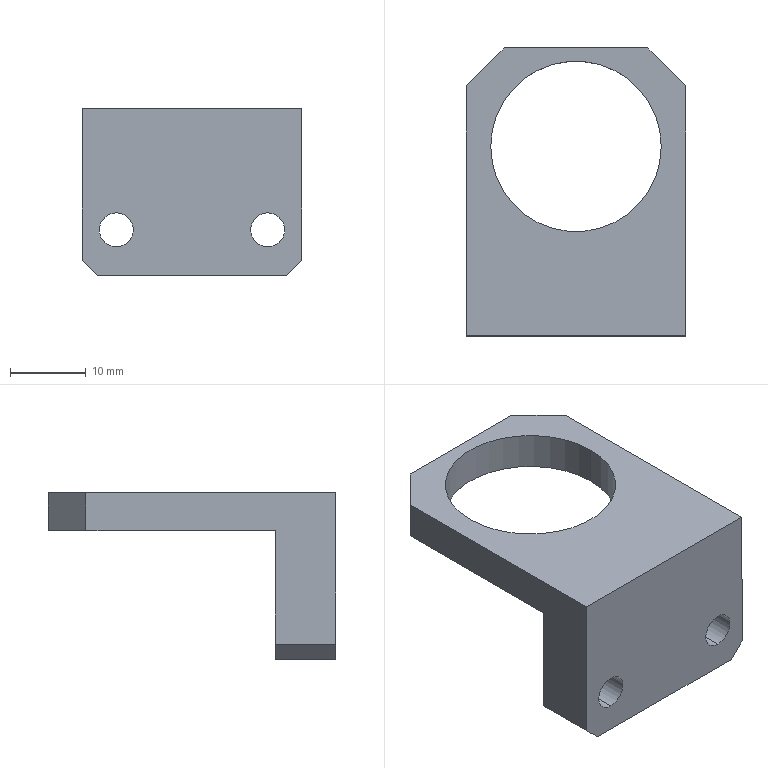Component | SolidWorks | F01AE00111-A2000-21TopEdgeAssembly-1_F01AE00111-A2055-1 | 1 solid | 18 faces | box 29 x 38 x 22 mm | volume 7054 mm3 | plane 12 | cylinder 6 | commonest cylinder face diameters 4.5 x4 22.5 x2
build123d program:
from build123d import *

# Parameters (mm, degrees)
SKETCH1_W           = 29
SKETCH1_H           = 38
BOSS_EXTRUDE1_DEPTH = 8
SKETCH2_W           = 22
SKETCH2_H           = 8
BOSS_EXTRUDE2_DEPTH = 29
SKETCH3_R           = 11.25
CUT_EXTRUDE1_DEPTH  = 12
CHAMFER1_SIZE       = 5
CHAMFER2_SIZE       = 2
SKETCH5_R           = 2.25
CUT_EXTRUDE3_DEPTH  = 12
SKETCH6_W           = 34.275
SKETCH6_H           = 35.36
CUT_EXTRUDE4_DEPTH  = 3


with BuildPart() as part:
    # Sketch1 → Boss-Extrude1 (new body)
    with BuildSketch(Plane.XY):
        Rectangle(SKETCH1_W, SKETCH1_H)
    extrude(amount=BOSS_EXTRUDE1_DEPTH)

    # Sketch2 → Boss-Extrude2 (add)
    with BuildSketch(Plane(origin=(14.5, 0, 0), x_dir=(0, 0, -1), z_dir=(1, 0, 0))):
        with Locations((3, -15)):
            Rectangle(SKETCH2_W, SKETCH2_H)
    extrude(amount=-BOSS_EXTRUDE2_DEPTH)

    # Sketch3 → Cut-Extrude1 (cut)
    with BuildSketch(Plane(origin=(0, 0, 0), x_dir=(-1, 0, 0), z_dir=(0, 0, -1))):
        with Locations((0, 6)):
            Circle(SKETCH3_R)
    extrude(amount=-CUT_EXTRUDE1_DEPTH, mode=Mode.SUBTRACT)

    # Chamfer1
    chamfer1_edges = [part.edges().sort_by_distance(p)[0] for p in [
        (-14.5, 19, 4),
        (14.5, 19, 4),
    ]]
    chamfer(chamfer1_edges, length=CHAMFER1_SIZE)

    # Chamfer2
    chamfer2_edges = [part.edges().sort_by_distance(p)[0] for p in [
        (14.5, -15, -14),
        (-14.5, -15, -14),
    ]]
    chamfer(chamfer2_edges, length=CHAMFER2_SIZE)

    # Sketch5 → Cut-Extrude3 (cut)
    with BuildSketch(Plane(origin=(0, -11, 0), x_dir=(1, 0, 0), z_dir=(0, 1, 0))):
        with Locations(Location((-10, 8, 0), (0, 0, 270))):
            Circle(SKETCH5_R)
        with Locations(Location((10, 8, 0), (0, 0, 270))):
            Circle(SKETCH5_R)
    extrude(amount=-CUT_EXTRUDE3_DEPTH, mode=Mode.SUBTRACT)

    # Sketch6 → Cut-Extrude4 (cut)
    with BuildSketch(Plane(origin=(0, 0, 0), x_dir=(-1, 0, 0), z_dir=(0, 0, -1))):
        with Locations((2.637, 6.68)):
            Rectangle(SKETCH6_W, SKETCH6_H)
    extrude(amount=-CUT_EXTRUDE4_DEPTH, mode=Mode.SUBTRACT)


solid = part.part

# Placed as in the assembly
solid = solid.moved(Location((-109.352, 76.548, -339.975), (0, 0, 0)))
STEP:
#1=CARTESIAN_POINT('',(-3.911,2.266,-13.788));
#2=VERTEX_POINT('',#1);
#3=CARTESIAN_POINT('',(-3.911,2.266,-13.611));
#4=VERTEX_POINT('',#3);
#5=CARTESIAN_POINT('',(-3.911,2.266,-13.7));
#6=DIRECTION('',(0.,1.,0.));
#7=DIRECTION('',(0.,0.,1.));
#8=AXIS2_PLACEMENT_3D('',#5,#6,#7);
#9=CIRCLE('',#8,0.08858);
#10=EDGE_CURVE('',#2,#4,#9,.T.);
#11=ORIENTED_EDGE('',*,*,#10,.F.);
#12=CARTESIAN_POINT('',(-3.911,2.581,-13.788));
#13=VERTEX_POINT('',#12);
#14=CARTESIAN_POINT('',(-3.911,2.108,-13.788));
#15=DIRECTION('',(0.,1.,0.));
#16=VECTOR('',#15,39.37);
#17=LINE('',#14,#16);
#18=EDGE_CURVE('',#2,#13,#17,.T.);
#19=ORIENTED_EDGE('',*,*,#18,.T.);
#20=CARTESIAN_POINT('',(-3.911,2.581,-13.611));
#21=VERTEX_POINT('',#20);
#22=CARTESIAN_POINT('',(-3.911,2.581,-13.7));
#23=DIRECTION('',(0.,1.,0.));
#24=DIRECTION('',(0.,0.,1.));
#25=AXIS2_PLACEMENT_3D('',#22,#23,#24);
#26=CIRCLE('',#25,0.08858);
#27=EDGE_CURVE('',#13,#21,#26,.T.);
#28=ORIENTED_EDGE('',*,*,#27,.T.);
#29=CARTESIAN_POINT('',(-3.911,2.108,-13.611));
#30=DIRECTION('',(0.,1.,0.));
#31=VECTOR('',#30,39.37);
#32=LINE('',#29,#31);
#33=EDGE_CURVE('',#4,#21,#32,.T.);
#34=ORIENTED_EDGE('',*,*,#33,.F.);
#35=EDGE_LOOP('',(#11,#19,#28,#34));
#36=FACE_OUTER_BOUND('',#35,.T.);
#37=CARTESIAN_POINT('',(-3.911,2.108,-13.7));
#38=DIRECTION('',(0.,1.,0.));
#39=DIRECTION('',(0.,0.,1.));
#40=AXIS2_PLACEMENT_3D('',#37,#38,#39);
#41=CYLINDRICAL_SURFACE('',#40,0.08858);
#42=ADVANCED_FACE('',(#36),#41,.F.);
#43=CARTESIAN_POINT('',(-4.699,2.266,-13.788));
#44=VERTEX_POINT('',#43);
#45=CARTESIAN_POINT('',(-4.699,2.266,-13.611));
#46=VERTEX_POINT('',#45);
#47=CARTESIAN_POINT('',(-4.699,2.266,-13.7));
#48=DIRECTION('',(0.,1.,0.));
#49=DIRECTION('',(0.,0.,1.));
#50=AXIS2_PLACEMENT_3D('',#47,#48,#49);
#51=CIRCLE('',#50,0.08858);
#52=EDGE_CURVE('',#44,#46,#51,.T.);
#53=ORIENTED_EDGE('',*,*,#52,.F.);
#54=CARTESIAN_POINT('',(-4.699,2.581,-13.788));
#55=VERTEX_POINT('',#54);
#56=CARTESIAN_POINT('',(-4.699,2.108,-13.788));
#57=DIRECTION('',(0.,1.,0.));
#58=VECTOR('',#57,39.37);
#59=LINE('',#56,#58);
#60=EDGE_CURVE('',#44,#55,#59,.T.);
#61=ORIENTED_EDGE('',*,*,#60,.T.);
#62=CARTESIAN_POINT('',(-4.699,2.581,-13.611));
#63=VERTEX_POINT('',#62);
#64=CARTESIAN_POINT('',(-4.699,2.581,-13.7));
#65=DIRECTION('',(0.,1.,0.));
#66=DIRECTION('',(0.,0.,1.));
#67=AXIS2_PLACEMENT_3D('',#64,#65,#66);
#68=CIRCLE('',#67,0.08858);
#69=EDGE_CURVE('',#55,#63,#68,.T.);
#70=ORIENTED_EDGE('',*,*,#69,.T.);
#71=CARTESIAN_POINT('',(-4.699,2.108,-13.611));
#72=DIRECTION('',(0.,1.,0.));
#73=VECTOR('',#72,39.37);
#74=LINE('',#71,#73);
#75=EDGE_CURVE('',#46,#63,#74,.T.);
#76=ORIENTED_EDGE('',*,*,#75,.F.);
#77=EDGE_LOOP('',(#53,#61,#70,#76));
#78=FACE_OUTER_BOUND('',#77,.T.);
#79=CARTESIAN_POINT('',(-4.699,2.108,-13.7));
#80=DIRECTION('',(0.,1.,0.));
#81=DIRECTION('',(0.,0.,1.));
#82=AXIS2_PLACEMENT_3D('',#79,#80,#81);
#83=CYLINDRICAL_SURFACE('',#82,0.08858);
#84=ADVANCED_FACE('',(#78),#83,.F.);
#85=CARTESIAN_POINT('',(-3.862,3.25,-13.07));
#86=VERTEX_POINT('',#85);
#87=CARTESIAN_POINT('',(-4.748,3.25,-13.07));
#88=VERTEX_POINT('',#87);
#89=CARTESIAN_POINT('',(-4.305,3.25,-13.07));
#90=DIRECTION('',(0.,0.,-1.));
#91=DIRECTION('',(-1.,0.,0.));
#92=AXIS2_PLACEMENT_3D('',#89,#90,#91);
#93=CIRCLE('',#92,0.4429);
#94=EDGE_CURVE('',#86,#88,#93,.T.);
#95=ORIENTED_EDGE('',*,*,#94,.F.);
#96=CARTESIAN_POINT('',(-3.862,3.25,-13.267));
#97=VERTEX_POINT('',#96);
#98=CARTESIAN_POINT('',(-3.862,3.25,-12.912));
#99=DIRECTION('',(0.,0.,-1.));
#100=VECTOR('',#99,39.37);
#101=LINE('',#98,#100);
#102=EDGE_CURVE('',#86,#97,#101,.T.);
#103=ORIENTED_EDGE('',*,*,#102,.T.);
#104=CARTESIAN_POINT('',(-4.748,3.25,-13.267));
#105=VERTEX_POINT('',#104);
#106=CARTESIAN_POINT('',(-4.305,3.25,-13.267));
#107=DIRECTION('',(0.,0.,-1.));
#108=DIRECTION('',(1.,0.,0.));
#109=AXIS2_PLACEMENT_3D('',#106,#107,#108);
#110=CIRCLE('',#109,0.4429);
#111=EDGE_CURVE('',#97,#105,#110,.T.);
#112=ORIENTED_EDGE('',*,*,#111,.T.);
#113=CARTESIAN_POINT('',(-4.748,3.25,-12.912));
#114=DIRECTION('',(0.,0.,-1.));
#115=VECTOR('',#114,39.37);
#116=LINE('',#113,#115);
#117=EDGE_CURVE('',#88,#105,#116,.T.);
#118=ORIENTED_EDGE('',*,*,#117,.F.);
#119=EDGE_LOOP('',(#95,#103,#112,#118));
#120=FACE_OUTER_BOUND('',#119,.T.);
#121=CARTESIAN_POINT('',(-4.305,3.25,-12.912));
#122=DIRECTION('',(0.,0.,-1.));
#123=DIRECTION('',(-1.,0.,0.));
#124=AXIS2_PLACEMENT_3D('',#121,#122,#123);
#125=CYLINDRICAL_SURFACE('',#124,0.4429);
#126=ADVANCED_FACE('',(#120),#125,.F.);
#127=CARTESIAN_POINT('',(-3.734,2.581,-13.857));
#128=VERTEX_POINT('',#127);
#129=CARTESIAN_POINT('',(-3.734,2.581,-13.267));
#130=VERTEX_POINT('',#129);
#131=CARTESIAN_POINT('',(-3.734,2.581,-13.07));
#132=DIRECTION('',(0.,0.,1.));
#133=VECTOR('',#132,39.37);
#134=LINE('',#131,#133);
#135=EDGE_CURVE('',#128,#130,#134,.T.);
#136=ORIENTED_EDGE('',*,*,#135,.T.);
#137=CARTESIAN_POINT('',(-3.734,3.565,-13.267));
#138=VERTEX_POINT('',#137);
#139=CARTESIAN_POINT('',(-3.734,2.581,-13.267));
#140=DIRECTION('',(0.,-1.,0.));
#141=VECTOR('',#140,39.37);
#142=LINE('',#139,#141);
#143=EDGE_CURVE('',#138,#130,#142,.T.);
#144=ORIENTED_EDGE('',*,*,#143,.F.);
#145=CARTESIAN_POINT('',(-3.734,3.565,-13.07));
#146=VERTEX_POINT('',#145);
#147=CARTESIAN_POINT('',(-3.734,3.565,-13.07));
#148=DIRECTION('',(0.,0.,1.));
#149=VECTOR('',#148,39.37);
#150=LINE('',#147,#149);
#151=EDGE_CURVE('',#138,#146,#150,.T.);
#152=ORIENTED_EDGE('',*,*,#151,.T.);
#153=CARTESIAN_POINT('',(-3.734,2.266,-13.07));
#154=VERTEX_POINT('',#153);
#155=CARTESIAN_POINT('',(-3.734,2.266,-13.07));
#156=DIRECTION('',(0.,1.,0.));
#157=VECTOR('',#156,39.37);
#158=LINE('',#155,#157);
#159=EDGE_CURVE('',#154,#146,#158,.T.);
#160=ORIENTED_EDGE('',*,*,#159,.F.);
#161=CARTESIAN_POINT('',(-3.734,2.266,-13.857));
#162=VERTEX_POINT('',#161);
#163=CARTESIAN_POINT('',(-3.734,2.266,-13.07));
#164=DIRECTION('',(0.,0.,-1.));
#165=VECTOR('',#164,39.37);
#166=LINE('',#163,#165);
#167=EDGE_CURVE('',#154,#162,#166,.T.);
#168=ORIENTED_EDGE('',*,*,#167,.T.);
#169=CARTESIAN_POINT('',(-3.734,2.581,-13.857));
#170=DIRECTION('',(0.,1.,0.));
#171=VECTOR('',#170,39.37);
#172=LINE('',#169,#171);
#173=EDGE_CURVE('',#162,#128,#172,.T.);
#174=ORIENTED_EDGE('',*,*,#173,.T.);
#175=EDGE_LOOP('',(#136,#144,#152,#160,#168,#174));
#176=FACE_OUTER_BOUND('',#175,.T.);
#177=CARTESIAN_POINT('',(-3.734,2.266,-13.07));
#178=DIRECTION('',(-1.,0.,0.));
#179=DIRECTION('',(0.,0.,1.));
#180=AXIS2_PLACEMENT_3D('',#177,#178,#179);
#181=PLANE('',#180);
#182=ADVANCED_FACE('',(#176),#181,.F.);
#183=CARTESIAN_POINT('',(-3.931,3.762,-13.07));
#184=VERTEX_POINT('',#183);
#185=CARTESIAN_POINT('',(-3.931,3.762,-13.267));
#186=VERTEX_POINT('',#185);
#187=CARTESIAN_POINT('',(-3.931,3.762,-13.07));
#188=DIRECTION('',(0.,0.,-1.));
#189=VECTOR('',#188,39.37);
#190=LINE('',#187,#189);
#191=EDGE_CURVE('',#184,#186,#190,.T.);
#192=ORIENTED_EDGE('',*,*,#191,.T.);
#193=CARTESIAN_POINT('',(-4.679,3.762,-13.267));
#194=VERTEX_POINT('',#193);
#195=CARTESIAN_POINT('',(-4.876,3.762,-13.267));
#196=DIRECTION('',(-1.,0.,0.));
#197=VECTOR('',#196,39.37);
#198=LINE('',#195,#197);
#199=EDGE_CURVE('',#186,#194,#198,.T.);
#200=ORIENTED_EDGE('',*,*,#199,.T.);
#201=CARTESIAN_POINT('',(-4.679,3.762,-13.07));
#202=VERTEX_POINT('',#201);
#203=CARTESIAN_POINT('',(-4.679,3.762,-13.07));
#204=DIRECTION('',(0.,0.,1.));
#205=VECTOR('',#204,39.37);
#206=LINE('',#203,#205);
#207=EDGE_CURVE('',#194,#202,#206,.T.);
#208=ORIENTED_EDGE('',*,*,#207,.T.);
#209=CARTESIAN_POINT('',(-4.876,3.762,-13.07));
#210=DIRECTION('',(-1.,0.,0.));
#211=VECTOR('',#210,39.37);
#212=LINE('',#209,#211);
#213=EDGE_CURVE('',#184,#202,#212,.T.);
#214=ORIENTED_EDGE('',*,*,#213,.F.);
#215=EDGE_LOOP('',(#192,#200,#208,#214));
#216=FACE_OUTER_BOUND('',#215,.T.);
#217=CARTESIAN_POINT('',(-4.876,3.762,-13.07));
#218=DIRECTION('',(0.,-1.,0.));
#219=DIRECTION('',(0.,0.,-1.));
#220=AXIS2_PLACEMENT_3D('',#217,#218,#219);
#221=PLANE('',#220);
#222=ADVANCED_FACE('',(#216),#221,.F.);
#223=CARTESIAN_POINT('',(-4.876,3.565,-13.267));
#224=VERTEX_POINT('',#223);
#225=CARTESIAN_POINT('',(-4.876,2.581,-13.267));
#226=VERTEX_POINT('',#225);
#227=CARTESIAN_POINT('',(-4.876,2.266,-13.267));
#228=DIRECTION('',(0.,-1.,0.));
#229=VECTOR('',#228,39.37);
#230=LINE('',#227,#229);
#231=EDGE_CURVE('',#224,#226,#230,.T.);
#232=ORIENTED_EDGE('',*,*,#231,.T.);
#233=CARTESIAN_POINT('',(-4.876,2.581,-13.857));
#234=VERTEX_POINT('',#233);
#235=CARTESIAN_POINT('',(-4.876,2.581,-13.07));
#236=DIRECTION('',(0.,0.,-1.));
#237=VECTOR('',#236,39.37);
#238=LINE('',#235,#237);
#239=EDGE_CURVE('',#226,#234,#238,.T.);
#240=ORIENTED_EDGE('',*,*,#239,.T.);
#241=CARTESIAN_POINT('',(-4.876,2.266,-13.857));
#242=VERTEX_POINT('',#241);
#243=CARTESIAN_POINT('',(-4.876,2.266,-13.857));
#244=DIRECTION('',(0.,-1.,0.));
#245=VECTOR('',#244,39.37);
#246=LINE('',#243,#245);
#247=EDGE_CURVE('',#234,#242,#246,.T.);
#248=ORIENTED_EDGE('',*,*,#247,.T.);
#249=CARTESIAN_POINT('',(-4.876,2.266,-13.07));
#250=VERTEX_POINT('',#249);
#251=CARTESIAN_POINT('',(-4.876,2.266,-13.07));
#252=DIRECTION('',(0.,0.,-1.));
#253=VECTOR('',#252,39.37);
#254=LINE('',#251,#253);
#255=EDGE_CURVE('',#250,#242,#254,.T.);
#256=ORIENTED_EDGE('',*,*,#255,.F.);
#257=CARTESIAN_POINT('',(-4.876,3.565,-13.07));
#258=VERTEX_POINT('',#257);
#259=CARTESIAN_POINT('',(-4.876,2.266,-13.07));
#260=DIRECTION('',(0.,-1.,0.));
#261=VECTOR('',#260,39.37);
#262=LINE('',#259,#261);
#263=EDGE_CURVE('',#258,#250,#262,.T.);
#264=ORIENTED_EDGE('',*,*,#263,.F.);
#265=CARTESIAN_POINT('',(-4.876,3.565,-13.07));
#266=DIRECTION('',(0.,0.,-1.));
#267=VECTOR('',#266,39.37);
#268=LINE('',#265,#267);
#269=EDGE_CURVE('',#258,#224,#268,.T.);
#270=ORIENTED_EDGE('',*,*,#269,.T.);
#271=EDGE_LOOP('',(#232,#240,#248,#256,#264,#270));
#272=FACE_OUTER_BOUND('',#271,.T.);
#273=CARTESIAN_POINT('',(-4.876,2.266,-13.07));
#274=DIRECTION('',(1.,0.,0.));
#275=DIRECTION('',(0.,0.,-1.));
#276=AXIS2_PLACEMENT_3D('',#273,#274,#275);
#277=PLANE('',#276);
#278=ADVANCED_FACE('',(#272),#277,.F.);
#279=CARTESIAN_POINT('',(-3.911,2.266,-13.7));
#280=DIRECTION('',(0.,1.,0.));
#281=DIRECTION('',(0.,0.,1.));
#282=AXIS2_PLACEMENT_3D('',#279,#280,#281);
#283=CIRCLE('',#282,0.08858);
#284=EDGE_CURVE('',#4,#2,#283,.T.);
#285=ORIENTED_EDGE('',*,*,#284,.T.);
#286=ORIENTED_EDGE('',*,*,#10,.T.);
#287=EDGE_LOOP('',(#285,#286));
#288=FACE_BOUND('',#287,.T.);
#289=CARTESIAN_POINT('',(-4.699,2.266,-13.7));
#290=DIRECTION('',(0.,1.,0.));
#291=DIRECTION('',(0.,0.,1.));
#292=AXIS2_PLACEMENT_3D('',#289,#290,#291);
#293=CIRCLE('',#292,0.08858);
#294=EDGE_CURVE('',#46,#44,#293,.T.);
#295=ORIENTED_EDGE('',*,*,#294,.T.);
#296=ORIENTED_EDGE('',*,*,#52,.T.);
#297=EDGE_LOOP('',(#295,#296));
#298=FACE_BOUND('',#297,.T.);
#299=ORIENTED_EDGE('',*,*,#255,.T.);
#300=CARTESIAN_POINT('',(-4.797,2.266,-13.936));
#301=VERTEX_POINT('',#300);
#302=CARTESIAN_POINT('',(-4.876,2.266,-13.857));
#303=DIRECTION('',(0.7071,0.,-0.7071));
#304=VECTOR('',#303,39.37);
#305=LINE('',#302,#304);
#306=EDGE_CURVE('',#242,#301,#305,.T.);
#307=ORIENTED_EDGE('',*,*,#306,.T.);
#308=CARTESIAN_POINT('',(-3.813,2.266,-13.936));
#309=VERTEX_POINT('',#308);
#310=CARTESIAN_POINT('',(-5.798,2.266,-13.936));
#311=DIRECTION('',(1.,0.,0.));
#312=VECTOR('',#311,39.37);
#313=LINE('',#310,#312);
#314=EDGE_CURVE('',#301,#309,#313,.T.);
#315=ORIENTED_EDGE('',*,*,#314,.T.);
#316=CARTESIAN_POINT('',(-3.734,2.266,-13.857));
#317=DIRECTION('',(0.7071,0.,0.7071));
#318=VECTOR('',#317,39.37);
#319=LINE('',#316,#318);
#320=EDGE_CURVE('',#309,#162,#319,.T.);
#321=ORIENTED_EDGE('',*,*,#320,.T.);
#322=ORIENTED_EDGE('',*,*,#167,.F.);
#323=CARTESIAN_POINT('',(-4.876,2.266,-13.07));
#324=DIRECTION('',(1.,0.,0.));
#325=VECTOR('',#324,39.37);
#326=LINE('',#323,#325);
#327=EDGE_CURVE('',#250,#154,#326,.T.);
#328=ORIENTED_EDGE('',*,*,#327,.F.);
#329=EDGE_LOOP('',(#299,#307,#315,#321,#322,#328));
#330=FACE_OUTER_BOUND('',#329,.T.);
#331=CARTESIAN_POINT('',(-4.876,2.266,-13.07));
#332=DIRECTION('',(0.,1.,0.));
#333=DIRECTION('',(0.,0.,1.));
#334=AXIS2_PLACEMENT_3D('',#331,#332,#333);
#335=PLANE('',#334);
#336=ADVANCED_FACE('',(#288,#298,#330),#335,.F.);
#337=CARTESIAN_POINT('',(-4.305,3.25,-13.07));
#338=DIRECTION('',(0.,0.,-1.));
#339=DIRECTION('',(-1.,0.,0.));
#340=AXIS2_PLACEMENT_3D('',#337,#338,#339);
#341=CIRCLE('',#340,0.4429);
#342=EDGE_CURVE('',#88,#86,#341,.T.);
#343=ORIENTED_EDGE('',*,*,#342,.T.);
#344=ORIENTED_EDGE('',*,*,#94,.T.);
#345=EDGE_LOOP('',(#343,#344));
#346=FACE_BOUND('',#345,.T.);
#347=ORIENTED_EDGE('',*,*,#213,.T.);
#348=CARTESIAN_POINT('',(-4.876,3.565,-13.07));
#349=DIRECTION('',(-0.7071,-0.7071,0.));
#350=VECTOR('',#349,39.37);
#351=LINE('',#348,#350);
#352=EDGE_CURVE('',#202,#258,#351,.T.);
#353=ORIENTED_EDGE('',*,*,#352,.T.);
#354=ORIENTED_EDGE('',*,*,#263,.T.);
#355=ORIENTED_EDGE('',*,*,#327,.T.);
#356=ORIENTED_EDGE('',*,*,#159,.T.);
#357=CARTESIAN_POINT('',(-3.931,3.762,-13.07));
#358=DIRECTION('',(-0.7071,0.7071,0.));
#359=VECTOR('',#358,39.37);
#360=LINE('',#357,#359);
#361=EDGE_CURVE('',#146,#184,#360,.T.);
#362=ORIENTED_EDGE('',*,*,#361,.T.);
#363=EDGE_LOOP('',(#347,#353,#354,#355,#356,#362));
#364=FACE_OUTER_BOUND('',#363,.T.);
#365=CARTESIAN_POINT('',(-4.305,3.014,-13.07));
#366=DIRECTION('',(0.,0.,-1.));
#367=DIRECTION('',(-1.,0.,0.));
#368=AXIS2_PLACEMENT_3D('',#365,#366,#367);
#369=PLANE('',#368);
#370=ADVANCED_FACE('',(#346,#364),#369,.F.);
#371=CARTESIAN_POINT('',(-3.911,2.581,-13.7));
#372=DIRECTION('',(0.,1.,0.));
#373=DIRECTION('',(0.,0.,1.));
#374=AXIS2_PLACEMENT_3D('',#371,#372,#373);
#375=CIRCLE('',#374,0.08858);
#376=EDGE_CURVE('',#21,#13,#375,.T.);
#377=ORIENTED_EDGE('',*,*,#376,.F.);
#378=ORIENTED_EDGE('',*,*,#27,.F.);
#379=EDGE_LOOP('',(#377,#378));
#380=FACE_BOUND('',#379,.T.);
#381=CARTESIAN_POINT('',(-4.699,2.581,-13.7));
#382=DIRECTION('',(0.,1.,0.));
#383=DIRECTION('',(0.,0.,1.));
#384=AXIS2_PLACEMENT_3D('',#381,#382,#383);
#385=CIRCLE('',#384,0.08858);
#386=EDGE_CURVE('',#63,#55,#385,.T.);
#387=ORIENTED_EDGE('',*,*,#386,.F.);
#388=ORIENTED_EDGE('',*,*,#69,.F.);
#389=EDGE_LOOP('',(#387,#388));
#390=FACE_BOUND('',#389,.T.);
#391=CARTESIAN_POINT('',(-4.797,2.581,-13.936));
#392=VERTEX_POINT('',#391);
#393=CARTESIAN_POINT('',(-3.813,2.581,-13.936));
#394=VERTEX_POINT('',#393);
#395=CARTESIAN_POINT('',(-5.798,2.581,-13.936));
#396=DIRECTION('',(1.,0.,0.));
#397=VECTOR('',#396,39.37);
#398=LINE('',#395,#397);
#399=EDGE_CURVE('',#392,#394,#398,.T.);
#400=ORIENTED_EDGE('',*,*,#399,.F.);
#401=CARTESIAN_POINT('',(-5.731,2.581,-13.003));
#402=DIRECTION('',(-0.7071,0.,0.7071));
#403=VECTOR('',#402,39.37);
#404=LINE('',#401,#403);
#405=EDGE_CURVE('',#392,#234,#404,.T.);
#406=ORIENTED_EDGE('',*,*,#405,.T.);
#407=ORIENTED_EDGE('',*,*,#239,.F.);
#408=CARTESIAN_POINT('',(-3.734,2.581,-13.267));
#409=DIRECTION('',(-1.,0.,0.));
#410=VECTOR('',#409,39.37);
#411=LINE('',#408,#410);
#412=EDGE_CURVE('',#130,#226,#411,.T.);
#413=ORIENTED_EDGE('',*,*,#412,.F.);
#414=ORIENTED_EDGE('',*,*,#135,.F.);
#415=CARTESIAN_POINT('',(-4.372,2.581,-14.495));
#416=DIRECTION('',(-0.7071,0.,-0.7071));
#417=VECTOR('',#416,39.37);
#418=LINE('',#415,#417);
#419=EDGE_CURVE('',#128,#394,#418,.T.);
#420=ORIENTED_EDGE('',*,*,#419,.T.);
#421=EDGE_LOOP('',(#400,#406,#407,#413,#414,#420));
#422=FACE_OUTER_BOUND('',#421,.T.);
#423=CARTESIAN_POINT('',(-5.798,2.581,-13.07));
#424=DIRECTION('',(0.,1.,0.));
#425=DIRECTION('',(0.,0.,1.));
#426=AXIS2_PLACEMENT_3D('',#423,#424,#425);
#427=PLANE('',#426);
#428=ADVANCED_FACE('',(#380,#390,#422),#427,.T.);
#429=ORIENTED_EDGE('',*,*,#314,.F.);
#430=CARTESIAN_POINT('',(-4.797,2.581,-13.936));
#431=DIRECTION('',(0.,1.,0.));
#432=VECTOR('',#431,39.37);
#433=LINE('',#430,#432);
#434=EDGE_CURVE('',#301,#392,#433,.T.);
#435=ORIENTED_EDGE('',*,*,#434,.T.);
#436=ORIENTED_EDGE('',*,*,#399,.T.);
#437=CARTESIAN_POINT('',(-3.813,2.266,-13.936));
#438=DIRECTION('',(0.,-1.,0.));
#439=VECTOR('',#438,39.37);
#440=LINE('',#437,#439);
#441=EDGE_CURVE('',#394,#309,#440,.T.);
#442=ORIENTED_EDGE('',*,*,#441,.T.);
#443=EDGE_LOOP('',(#429,#435,#436,#442));
#444=FACE_OUTER_BOUND('',#443,.T.);
#445=CARTESIAN_POINT('',(-5.798,2.266,-13.936));
#446=DIRECTION('',(0.,0.,-1.));
#447=DIRECTION('',(-1.,0.,0.));
#448=AXIS2_PLACEMENT_3D('',#445,#446,#447);
#449=PLANE('',#448);
#450=ADVANCED_FACE('',(#444),#449,.T.);
#451=ORIENTED_EDGE('',*,*,#102,.F.);
#452=ORIENTED_EDGE('',*,*,#342,.F.);
#453=ORIENTED_EDGE('',*,*,#117,.T.);
#454=CARTESIAN_POINT('',(-4.305,3.25,-13.267));
#455=DIRECTION('',(0.,0.,-1.));
#456=DIRECTION('',(1.,0.,0.));
#457=AXIS2_PLACEMENT_3D('',#454,#455,#456);
#458=CIRCLE('',#457,0.4429);
#459=EDGE_CURVE('',#105,#97,#458,.T.);
#460=ORIENTED_EDGE('',*,*,#459,.T.);
#461=EDGE_LOOP('',(#451,#452,#453,#460));
#462=FACE_OUTER_BOUND('',#461,.T.);
#463=CARTESIAN_POINT('',(-4.305,3.25,-12.912));
#464=DIRECTION('',(0.,0.,-1.));
#465=DIRECTION('',(-1.,0.,0.));
#466=AXIS2_PLACEMENT_3D('',#463,#464,#465);
#467=CYLINDRICAL_SURFACE('',#466,0.4429);
#468=ADVANCED_FACE('',(#462),#467,.F.);
#469=CARTESIAN_POINT('',(-4.876,3.565,-13.267));
#470=DIRECTION('',(0.7071,0.7071,0.));
#471=VECTOR('',#470,39.37);
#472=LINE('',#469,#471);
#473=EDGE_CURVE('',#224,#194,#472,.T.);
#474=ORIENTED_EDGE('',*,*,#473,.F.);
#475=ORIENTED_EDGE('',*,*,#269,.F.);
#476=ORIENTED_EDGE('',*,*,#352,.F.);
#477=ORIENTED_EDGE('',*,*,#207,.F.);
#478=EDGE_LOOP('',(#474,#475,#476,#477));
#479=FACE_OUTER_BOUND('',#478,.T.);
#480=CARTESIAN_POINT('',(-4.876,3.565,-13.07));
#481=DIRECTION('',(0.7071,-0.7071,0.));
#482=DIRECTION('',(0.,0.,-1.));
#483=AXIS2_PLACEMENT_3D('',#480,#481,#482);
#484=PLANE('',#483);
#485=ADVANCED_FACE('',(#479),#484,.F.);
#486=CARTESIAN_POINT('',(-3.931,3.762,-13.267));
#487=DIRECTION('',(0.7071,-0.7071,0.));
#488=VECTOR('',#487,39.37);
#489=LINE('',#486,#488);
#490=EDGE_CURVE('',#186,#138,#489,.T.);
#491=ORIENTED_EDGE('',*,*,#490,.F.);
#492=ORIENTED_EDGE('',*,*,#191,.F.);
#493=ORIENTED_EDGE('',*,*,#361,.F.);
#494=ORIENTED_EDGE('',*,*,#151,.F.);
#495=EDGE_LOOP('',(#491,#492,#493,#494));
#496=FACE_OUTER_BOUND('',#495,.T.);
#497=CARTESIAN_POINT('',(-3.931,3.762,-13.07));
#498=DIRECTION('',(-0.7071,-0.7071,0.));
#499=DIRECTION('',(0.,0.,-1.));
#500=AXIS2_PLACEMENT_3D('',#497,#498,#499);
#501=PLANE('',#500);
#502=ADVANCED_FACE('',(#496),#501,.F.);
#503=ORIENTED_EDGE('',*,*,#405,.F.);
#504=ORIENTED_EDGE('',*,*,#434,.F.);
#505=ORIENTED_EDGE('',*,*,#306,.F.);
#506=ORIENTED_EDGE('',*,*,#247,.F.);
#507=EDGE_LOOP('',(#503,#504,#505,#506));
#508=FACE_OUTER_BOUND('',#507,.T.);
#509=CARTESIAN_POINT('',(-4.876,2.266,-13.857));
#510=DIRECTION('',(-0.7071,0.,-0.7071));
#511=DIRECTION('',(0.,1.,0.));
#512=AXIS2_PLACEMENT_3D('',#509,#510,#511);
#513=PLANE('',#512);
#514=ADVANCED_FACE('',(#508),#513,.T.);
#515=ORIENTED_EDGE('',*,*,#320,.F.);
#516=ORIENTED_EDGE('',*,*,#441,.F.);
#517=ORIENTED_EDGE('',*,*,#419,.F.);
#518=ORIENTED_EDGE('',*,*,#173,.F.);
#519=EDGE_LOOP('',(#515,#516,#517,#518));
#520=FACE_OUTER_BOUND('',#519,.T.);
#521=CARTESIAN_POINT('',(-3.734,2.266,-13.857));
#522=DIRECTION('',(0.7071,0.,-0.7071));
#523=DIRECTION('',(0.,-1.,0.));
#524=AXIS2_PLACEMENT_3D('',#521,#522,#523);
#525=PLANE('',#524);
#526=ADVANCED_FACE('',(#520),#525,.T.);
#527=ORIENTED_EDGE('',*,*,#60,.F.);
#528=ORIENTED_EDGE('',*,*,#294,.F.);
#529=ORIENTED_EDGE('',*,*,#75,.T.);
#530=ORIENTED_EDGE('',*,*,#386,.T.);
#531=EDGE_LOOP('',(#527,#528,#529,#530));
#532=FACE_OUTER_BOUND('',#531,.T.);
#533=CARTESIAN_POINT('',(-4.699,2.108,-13.7));
#534=DIRECTION('',(0.,1.,0.));
#535=DIRECTION('',(0.,0.,1.));
#536=AXIS2_PLACEMENT_3D('',#533,#534,#535);
#537=CYLINDRICAL_SURFACE('',#536,0.08858);
#538=ADVANCED_FACE('',(#532),#537,.F.);
#539=ORIENTED_EDGE('',*,*,#18,.F.);
#540=ORIENTED_EDGE('',*,*,#284,.F.);
#541=ORIENTED_EDGE('',*,*,#33,.T.);
#542=ORIENTED_EDGE('',*,*,#376,.T.);
#543=EDGE_LOOP('',(#539,#540,#541,#542));
#544=FACE_OUTER_BOUND('',#543,.T.);
#545=CARTESIAN_POINT('',(-3.911,2.108,-13.7));
#546=DIRECTION('',(0.,1.,0.));
#547=DIRECTION('',(0.,0.,1.));
#548=AXIS2_PLACEMENT_3D('',#545,#546,#547);
#549=CYLINDRICAL_SURFACE('',#548,0.08858);
#550=ADVANCED_FACE('',(#544),#549,.F.);
#551=ORIENTED_EDGE('',*,*,#473,.T.);
#552=ORIENTED_EDGE('',*,*,#199,.F.);
#553=ORIENTED_EDGE('',*,*,#490,.T.);
#554=ORIENTED_EDGE('',*,*,#143,.T.);
#555=ORIENTED_EDGE('',*,*,#412,.T.);
#556=ORIENTED_EDGE('',*,*,#231,.F.);
#557=EDGE_LOOP('',(#551,#552,#553,#554,#555,#556));
#558=FACE_OUTER_BOUND('',#557,.T.);
#559=ORIENTED_EDGE('',*,*,#459,.F.);
#560=ORIENTED_EDGE('',*,*,#111,.F.);
#561=EDGE_LOOP('',(#559,#560));
#562=FACE_BOUND('',#561,.T.);
#563=CARTESIAN_POINT('',(-4.305,3.014,-13.267));
#564=DIRECTION('',(0.,0.,1.));
#565=DIRECTION('',(1.,0.,0.));
#566=AXIS2_PLACEMENT_3D('',#563,#564,#565);
#567=PLANE('',#566);
#568=ADVANCED_FACE('',(#558,#562),#567,.F.);
#569=CLOSED_SHELL('',(#42,#84,#126,#182,#222,#278,#336,#370,#428,#450,#468,#485,#502,#514,#526,#538,#550,#568));
#570=MANIFOLD_SOLID_BREP('',#569);
#571=CARTESIAN_POINT('',(0.,0.,0.));
#572=DIRECTION('',(0.,0.,1.));
#573=DIRECTION('',(1.,0.,0.));
#574=AXIS2_PLACEMENT_3D('',#571,#572,#573);
#575=(LENGTH_UNIT()NAMED_UNIT(*)SI_UNIT($,.METRE.));
#576=LENGTH_MEASURE_WITH_UNIT(LENGTH_MEASURE(0.0254),#575);
#577=DIMENSIONAL_EXPONENTS(1.,0.,0.,0.,0.,0.,0.);
#578=(CONVERSION_BASED_UNIT('',#576)LENGTH_UNIT()NAMED_UNIT(#577));
#579=UNCERTAINTY_MEASURE_WITH_UNIT(LENGTH_MEASURE(0.00001),#578,'','');
#580=(NAMED_UNIT(*)PLANE_ANGLE_UNIT()SI_UNIT($,.RADIAN.));
#581=(NAMED_UNIT(*)SI_UNIT($,.STERADIAN.)SOLID_ANGLE_UNIT());
#582=(GEOMETRIC_REPRESENTATION_CONTEXT(3)GLOBAL_UNCERTAINTY_ASSIGNED_CONTEXT((#579))GLOBAL_UNIT_ASSIGNED_CONTEXT((#578,#580,#581))REPRESENTATION_CONTEXT('',''));
#583=ADVANCED_BREP_SHAPE_REPRESENTATION('',(#570,#574),#582);
#584=COLOUR_RGB('',0.7922,0.8196,0.9333);
#585=FILL_AREA_STYLE_COLOUR('',#584);
#586=FILL_AREA_STYLE('',(#585));
#587=SURFACE_STYLE_FILL_AREA(#586);
#588=SURFACE_SIDE_STYLE('',(#587));
#589=SURFACE_STYLE_USAGE(.BOTH.,#588);
#590=PRESENTATION_STYLE_ASSIGNMENT((#589));
#591=STYLED_ITEM('',(#590),#570);
#592=PRESENTATION_LAYER_ASSIGNMENT('','',(#591));
#593=(LENGTH_UNIT()NAMED_UNIT(*)SI_UNIT($,.METRE.));
#594=LENGTH_MEASURE_WITH_UNIT(LENGTH_MEASURE(0.0254),#593);
#595=DIMENSIONAL_EXPONENTS(1.,0.,0.,0.,0.,0.,0.);
#596=(CONVERSION_BASED_UNIT('',#594)LENGTH_UNIT()NAMED_UNIT(#595));
#597=UNCERTAINTY_MEASURE_WITH_UNIT(LENGTH_MEASURE(0.00001),#596,'','');
#598=(NAMED_UNIT(*)PLANE_ANGLE_UNIT()SI_UNIT($,.RADIAN.));
#599=(NAMED_UNIT(*)SI_UNIT($,.STERADIAN.)SOLID_ANGLE_UNIT());
#600=(GEOMETRIC_REPRESENTATION_CONTEXT(3)GLOBAL_UNCERTAINTY_ASSIGNED_CONTEXT((#597))GLOBAL_UNIT_ASSIGNED_CONTEXT((#596,#598,#599))REPRESENTATION_CONTEXT('',''));
#601=MECHANICAL_DESIGN_GEOMETRIC_PRESENTATION_REPRESENTATION('',(#591),#600);